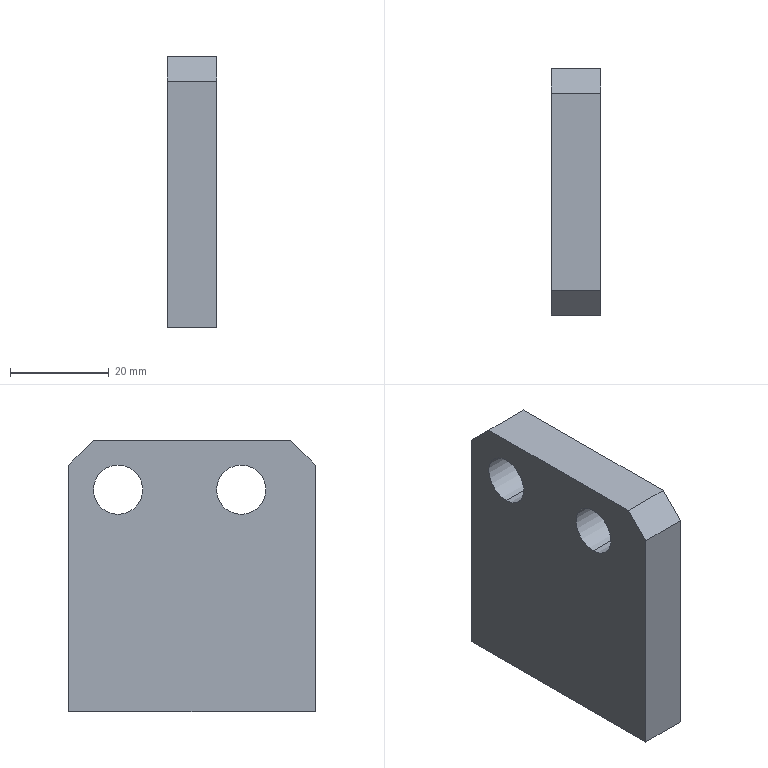Component | SolidWorks | 07-1 | 1 solid | 12 faces | box 10 x 50 x 55 mm | volume 25679 mm3 | plane 8 | cylinder 4 | commonest cylinder face diameters 10 x4
build123d program:
from build123d import *

# Parameters (mm, degrees)
SKETCH1_W           = 55
SKETCH1_H           = 50
SKETCH1_R           = 5
BOSS_EXTRUDE1_DEPTH = 10
CHAMFER1_SIZE       = 5


with BuildPart() as part:
    # Sketch1 → Boss-Extrude1 (new body)
    with BuildSketch(Plane.XY):
        with Locations((-21.5, 205)):
            Rectangle(SKETCH1_W, SKETCH1_H)
        with Locations((-39, 220)):
            Circle(SKETCH1_R, mode=Mode.SUBTRACT)
        with Locations((-39, 195)):
            Circle(SKETCH1_R, mode=Mode.SUBTRACT)
    extrude(amount=BOSS_EXTRUDE1_DEPTH)

    # Chamfer1
    chamfer1_edges = [part.edges().sort_by_distance(p)[0] for p in [
        (-49, 180, 5),
        (-49, 230, 5),
    ]]
    chamfer(chamfer1_edges, length=CHAMFER1_SIZE)


solid = part.part

# Placed as in the assembly
solid = solid.moved(Location((0, 0, 0), (0, 90, 0)))
STEP:
#1=COLOUR_RGB('',0.7922,0.8196,0.9333);
#2=FILL_AREA_STYLE_COLOUR('',#1);
#3=FILL_AREA_STYLE('',(#2));
#4=SURFACE_STYLE_FILL_AREA(#3);
#5=SURFACE_SIDE_STYLE('',(#4));
#6=SURFACE_STYLE_USAGE(.BOTH.,#5);
#7=PRESENTATION_STYLE_ASSIGNMENT((#6));
#8=CARTESIAN_POINT('',(0.3937,7.677,1.732));
#9=VERTEX_POINT('',#8);
#10=CARTESIAN_POINT('',(0.3937,7.677,1.339));
#11=VERTEX_POINT('',#10);
#12=CARTESIAN_POINT('',(0.3937,7.677,1.535));
#13=DIRECTION('',(1.,0.,0.));
#14=DIRECTION('',(0.,0.,-1.));
#15=AXIS2_PLACEMENT_3D('',#12,#13,#14);
#16=CIRCLE('',#15,0.1969);
#17=EDGE_CURVE('',#9,#11,#16,.T.);
#18=ORIENTED_EDGE('',*,*,#17,.T.);
#19=CARTESIAN_POINT('',(0.,7.677,1.339));
#20=VERTEX_POINT('',#19);
#21=CARTESIAN_POINT('',(0.3937,7.677,1.339));
#22=DIRECTION('',(-1.,0.,0.));
#23=VECTOR('',#22,39.37);
#24=LINE('',#21,#23);
#25=EDGE_CURVE('',#11,#20,#24,.T.);
#26=ORIENTED_EDGE('',*,*,#25,.T.);
#27=CARTESIAN_POINT('',(0.,7.677,1.732));
#28=VERTEX_POINT('',#27);
#29=CARTESIAN_POINT('',(0.,7.677,1.535));
#30=DIRECTION('',(1.,0.,0.));
#31=DIRECTION('',(0.,0.,-1.));
#32=AXIS2_PLACEMENT_3D('',#29,#30,#31);
#33=CIRCLE('',#32,0.1969);
#34=EDGE_CURVE('',#28,#20,#33,.T.);
#35=ORIENTED_EDGE('',*,*,#34,.F.);
#36=CARTESIAN_POINT('',(0.3937,7.677,1.732));
#37=DIRECTION('',(-1.,0.,0.));
#38=VECTOR('',#37,39.37);
#39=LINE('',#36,#38);
#40=EDGE_CURVE('',#9,#28,#39,.T.);
#41=ORIENTED_EDGE('',*,*,#40,.F.);
#42=EDGE_LOOP('',(#18,#26,#35,#41));
#43=FACE_OUTER_BOUND('',#42,.T.);
#44=CARTESIAN_POINT('',(0.3937,7.677,1.535));
#45=DIRECTION('',(-1.,0.,0.));
#46=DIRECTION('',(0.,0.,1.));
#47=AXIS2_PLACEMENT_3D('',#44,#45,#46);
#48=CYLINDRICAL_SURFACE('',#47,0.1969);
#49=ADVANCED_FACE('',(#43),#48,.F.);
#50=CARTESIAN_POINT('',(0.3937,8.661,1.732));
#51=VERTEX_POINT('',#50);
#52=CARTESIAN_POINT('',(0.3937,8.661,1.339));
#53=VERTEX_POINT('',#52);
#54=CARTESIAN_POINT('',(0.3937,8.661,1.535));
#55=DIRECTION('',(1.,0.,0.));
#56=DIRECTION('',(0.,0.,-1.));
#57=AXIS2_PLACEMENT_3D('',#54,#55,#56);
#58=CIRCLE('',#57,0.1969);
#59=EDGE_CURVE('',#51,#53,#58,.T.);
#60=ORIENTED_EDGE('',*,*,#59,.T.);
#61=CARTESIAN_POINT('',(0.,8.661,1.339));
#62=VERTEX_POINT('',#61);
#63=CARTESIAN_POINT('',(0.3937,8.661,1.339));
#64=DIRECTION('',(-1.,0.,0.));
#65=VECTOR('',#64,39.37);
#66=LINE('',#63,#65);
#67=EDGE_CURVE('',#53,#62,#66,.T.);
#68=ORIENTED_EDGE('',*,*,#67,.T.);
#69=CARTESIAN_POINT('',(0.,8.661,1.732));
#70=VERTEX_POINT('',#69);
#71=CARTESIAN_POINT('',(0.,8.661,1.535));
#72=DIRECTION('',(1.,0.,0.));
#73=DIRECTION('',(0.,0.,-1.));
#74=AXIS2_PLACEMENT_3D('',#71,#72,#73);
#75=CIRCLE('',#74,0.1969);
#76=EDGE_CURVE('',#70,#62,#75,.T.);
#77=ORIENTED_EDGE('',*,*,#76,.F.);
#78=CARTESIAN_POINT('',(0.3937,8.661,1.732));
#79=DIRECTION('',(-1.,0.,0.));
#80=VECTOR('',#79,39.37);
#81=LINE('',#78,#80);
#82=EDGE_CURVE('',#51,#70,#81,.T.);
#83=ORIENTED_EDGE('',*,*,#82,.F.);
#84=EDGE_LOOP('',(#60,#68,#77,#83));
#85=FACE_OUTER_BOUND('',#84,.T.);
#86=CARTESIAN_POINT('',(0.3937,8.661,1.535));
#87=DIRECTION('',(-1.,0.,0.));
#88=DIRECTION('',(0.,0.,1.));
#89=AXIS2_PLACEMENT_3D('',#86,#87,#88);
#90=CYLINDRICAL_SURFACE('',#89,0.1969);
#91=ADVANCED_FACE('',(#85),#90,.F.);
#92=CARTESIAN_POINT('',(0.3937,8.858,1.929));
#93=VERTEX_POINT('',#92);
#94=CARTESIAN_POINT('',(0.3937,7.283,1.929));
#95=VERTEX_POINT('',#94);
#96=CARTESIAN_POINT('',(0.3937,9.055,1.929));
#97=DIRECTION('',(0.,-1.,-0.));
#98=VECTOR('',#97,39.37);
#99=LINE('',#96,#98);
#100=EDGE_CURVE('',#93,#95,#99,.T.);
#101=ORIENTED_EDGE('',*,*,#100,.T.);
#102=CARTESIAN_POINT('',(0.3937,7.087,1.732));
#103=VERTEX_POINT('',#102);
#104=CARTESIAN_POINT('',(0.3937,7.087,1.732));
#105=DIRECTION('',(0.,-0.7071,-0.7071));
#106=VECTOR('',#105,39.37);
#107=LINE('',#104,#106);
#108=EDGE_CURVE('',#95,#103,#107,.T.);
#109=ORIENTED_EDGE('',*,*,#108,.T.);
#110=CARTESIAN_POINT('',(0.3937,7.087,-0.2362));
#111=VERTEX_POINT('',#110);
#112=CARTESIAN_POINT('',(0.3937,7.087,-0.2362));
#113=DIRECTION('',(0.,0.,-1.));
#114=VECTOR('',#113,39.37);
#115=LINE('',#112,#114);
#116=EDGE_CURVE('',#103,#111,#115,.T.);
#117=ORIENTED_EDGE('',*,*,#116,.T.);
#118=CARTESIAN_POINT('',(0.3937,9.055,-0.2362));
#119=VERTEX_POINT('',#118);
#120=CARTESIAN_POINT('',(0.3937,9.055,-0.2362));
#121=DIRECTION('',(0.,1.,0.));
#122=VECTOR('',#121,39.37);
#123=LINE('',#120,#122);
#124=EDGE_CURVE('',#111,#119,#123,.T.);
#125=ORIENTED_EDGE('',*,*,#124,.T.);
#126=CARTESIAN_POINT('',(0.3937,9.055,1.732));
#127=VERTEX_POINT('',#126);
#128=CARTESIAN_POINT('',(0.3937,9.055,-0.2362));
#129=DIRECTION('',(0.,0.,1.));
#130=VECTOR('',#129,39.37);
#131=LINE('',#128,#130);
#132=EDGE_CURVE('',#119,#127,#131,.T.);
#133=ORIENTED_EDGE('',*,*,#132,.T.);
#134=CARTESIAN_POINT('',(0.3937,8.858,1.929));
#135=DIRECTION('',(0.,-0.7071,0.7071));
#136=VECTOR('',#135,39.37);
#137=LINE('',#134,#136);
#138=EDGE_CURVE('',#127,#93,#137,.T.);
#139=ORIENTED_EDGE('',*,*,#138,.T.);
#140=EDGE_LOOP('',(#101,#109,#117,#125,#133,#139));
#141=FACE_OUTER_BOUND('',#140,.T.);
#142=ORIENTED_EDGE('',*,*,#59,.F.);
#143=CARTESIAN_POINT('',(0.3937,8.661,1.535));
#144=DIRECTION('',(1.,0.,0.));
#145=DIRECTION('',(0.,0.,-1.));
#146=AXIS2_PLACEMENT_3D('',#143,#144,#145);
#147=CIRCLE('',#146,0.1969);
#148=EDGE_CURVE('',#53,#51,#147,.T.);
#149=ORIENTED_EDGE('',*,*,#148,.F.);
#150=EDGE_LOOP('',(#142,#149));
#151=FACE_BOUND('',#150,.T.);
#152=ORIENTED_EDGE('',*,*,#17,.F.);
#153=CARTESIAN_POINT('',(0.3937,7.677,1.535));
#154=DIRECTION('',(1.,0.,0.));
#155=DIRECTION('',(0.,0.,-1.));
#156=AXIS2_PLACEMENT_3D('',#153,#154,#155);
#157=CIRCLE('',#156,0.1969);
#158=EDGE_CURVE('',#11,#9,#157,.T.);
#159=ORIENTED_EDGE('',*,*,#158,.F.);
#160=EDGE_LOOP('',(#152,#159));
#161=FACE_BOUND('',#160,.T.);
#162=CARTESIAN_POINT('',(0.3937,0.,0.));
#163=DIRECTION('',(-1.,0.,0.));
#164=DIRECTION('',(0.,0.,1.));
#165=AXIS2_PLACEMENT_3D('',#162,#163,#164);
#166=PLANE('',#165);
#167=ADVANCED_FACE('',(#141,#151,#161),#166,.F.);
#168=ORIENTED_EDGE('',*,*,#76,.T.);
#169=CARTESIAN_POINT('',(0.,8.661,1.535));
#170=DIRECTION('',(1.,0.,0.));
#171=DIRECTION('',(0.,0.,-1.));
#172=AXIS2_PLACEMENT_3D('',#169,#170,#171);
#173=CIRCLE('',#172,0.1969);
#174=EDGE_CURVE('',#62,#70,#173,.T.);
#175=ORIENTED_EDGE('',*,*,#174,.T.);
#176=EDGE_LOOP('',(#168,#175));
#177=FACE_BOUND('',#176,.T.);
#178=CARTESIAN_POINT('',(0.,7.087,1.732));
#179=VERTEX_POINT('',#178);
#180=CARTESIAN_POINT('',(0.,7.087,-0.2362));
#181=VERTEX_POINT('',#180);
#182=CARTESIAN_POINT('',(0.,7.087,-0.2362));
#183=DIRECTION('',(0.,0.,-1.));
#184=VECTOR('',#183,39.37);
#185=LINE('',#182,#184);
#186=EDGE_CURVE('',#179,#181,#185,.T.);
#187=ORIENTED_EDGE('',*,*,#186,.F.);
#188=CARTESIAN_POINT('',(0.,7.283,1.929));
#189=VERTEX_POINT('',#188);
#190=CARTESIAN_POINT('',(0.,2.677,-2.677));
#191=DIRECTION('',(0.,0.7071,0.7071));
#192=VECTOR('',#191,39.37);
#193=LINE('',#190,#192);
#194=EDGE_CURVE('',#179,#189,#193,.T.);
#195=ORIENTED_EDGE('',*,*,#194,.T.);
#196=CARTESIAN_POINT('',(0.,8.858,1.929));
#197=VERTEX_POINT('',#196);
#198=CARTESIAN_POINT('',(0.,9.055,1.929));
#199=DIRECTION('',(0.,-1.,-0.));
#200=VECTOR('',#199,39.37);
#201=LINE('',#198,#200);
#202=EDGE_CURVE('',#197,#189,#201,.T.);
#203=ORIENTED_EDGE('',*,*,#202,.F.);
#204=CARTESIAN_POINT('',(0.,9.055,1.732));
#205=VERTEX_POINT('',#204);
#206=CARTESIAN_POINT('',(0.,5.394,5.394));
#207=DIRECTION('',(0.,0.7071,-0.7071));
#208=VECTOR('',#207,39.37);
#209=LINE('',#206,#208);
#210=EDGE_CURVE('',#197,#205,#209,.T.);
#211=ORIENTED_EDGE('',*,*,#210,.T.);
#212=CARTESIAN_POINT('',(0.,9.055,-0.2362));
#213=VERTEX_POINT('',#212);
#214=CARTESIAN_POINT('',(0.,9.055,-0.2362));
#215=DIRECTION('',(0.,0.,1.));
#216=VECTOR('',#215,39.37);
#217=LINE('',#214,#216);
#218=EDGE_CURVE('',#213,#205,#217,.T.);
#219=ORIENTED_EDGE('',*,*,#218,.F.);
#220=CARTESIAN_POINT('',(0.,9.055,-0.2362));
#221=DIRECTION('',(0.,1.,0.));
#222=VECTOR('',#221,39.37);
#223=LINE('',#220,#222);
#224=EDGE_CURVE('',#181,#213,#223,.T.);
#225=ORIENTED_EDGE('',*,*,#224,.F.);
#226=EDGE_LOOP('',(#187,#195,#203,#211,#219,#225));
#227=FACE_OUTER_BOUND('',#226,.T.);
#228=ORIENTED_EDGE('',*,*,#34,.T.);
#229=CARTESIAN_POINT('',(0.,7.677,1.535));
#230=DIRECTION('',(1.,0.,0.));
#231=DIRECTION('',(0.,0.,-1.));
#232=AXIS2_PLACEMENT_3D('',#229,#230,#231);
#233=CIRCLE('',#232,0.1969);
#234=EDGE_CURVE('',#20,#28,#233,.T.);
#235=ORIENTED_EDGE('',*,*,#234,.T.);
#236=EDGE_LOOP('',(#228,#235));
#237=FACE_BOUND('',#236,.T.);
#238=CARTESIAN_POINT('',(0.,0.,0.));
#239=DIRECTION('',(-1.,0.,0.));
#240=DIRECTION('',(0.,0.,1.));
#241=AXIS2_PLACEMENT_3D('',#238,#239,#240);
#242=PLANE('',#241);
#243=ADVANCED_FACE('',(#177,#227,#237),#242,.T.);
#244=ORIENTED_EDGE('',*,*,#224,.T.);
#245=CARTESIAN_POINT('',(0.3937,9.055,-0.2362));
#246=DIRECTION('',(-1.,0.,0.));
#247=VECTOR('',#246,39.37);
#248=LINE('',#245,#247);
#249=EDGE_CURVE('',#119,#213,#248,.T.);
#250=ORIENTED_EDGE('',*,*,#249,.F.);
#251=ORIENTED_EDGE('',*,*,#124,.F.);
#252=CARTESIAN_POINT('',(0.3937,7.087,-0.2362));
#253=DIRECTION('',(-1.,0.,0.));
#254=VECTOR('',#253,39.37);
#255=LINE('',#252,#254);
#256=EDGE_CURVE('',#111,#181,#255,.T.);
#257=ORIENTED_EDGE('',*,*,#256,.T.);
#258=EDGE_LOOP('',(#244,#250,#251,#257));
#259=FACE_OUTER_BOUND('',#258,.T.);
#260=CARTESIAN_POINT('',(0.3937,9.055,-0.2362));
#261=DIRECTION('',(0.,-0.,1.));
#262=DIRECTION('',(0.,-1.,-0.));
#263=AXIS2_PLACEMENT_3D('',#260,#261,#262);
#264=PLANE('',#263);
#265=ADVANCED_FACE('',(#259),#264,.F.);
#266=ORIENTED_EDGE('',*,*,#218,.T.);
#267=CARTESIAN_POINT('',(0.3937,9.055,1.732));
#268=DIRECTION('',(1.,0.,0.));
#269=VECTOR('',#268,39.37);
#270=LINE('',#267,#269);
#271=EDGE_CURVE('',#205,#127,#270,.T.);
#272=ORIENTED_EDGE('',*,*,#271,.T.);
#273=ORIENTED_EDGE('',*,*,#132,.F.);
#274=ORIENTED_EDGE('',*,*,#249,.T.);
#275=EDGE_LOOP('',(#266,#272,#273,#274));
#276=FACE_OUTER_BOUND('',#275,.T.);
#277=CARTESIAN_POINT('',(0.3937,9.055,-0.2362));
#278=DIRECTION('',(0.,-1.,0.));
#279=DIRECTION('',(0.,-0.,-1.));
#280=AXIS2_PLACEMENT_3D('',#277,#278,#279);
#281=PLANE('',#280);
#282=ADVANCED_FACE('',(#276),#281,.F.);
#283=ORIENTED_EDGE('',*,*,#202,.T.);
#284=CARTESIAN_POINT('',(0.3937,7.283,1.929));
#285=DIRECTION('',(1.,0.,0.));
#286=VECTOR('',#285,39.37);
#287=LINE('',#284,#286);
#288=EDGE_CURVE('',#189,#95,#287,.T.);
#289=ORIENTED_EDGE('',*,*,#288,.T.);
#290=ORIENTED_EDGE('',*,*,#100,.F.);
#291=CARTESIAN_POINT('',(0.3937,8.858,1.929));
#292=DIRECTION('',(-1.,0.,0.));
#293=VECTOR('',#292,39.37);
#294=LINE('',#291,#293);
#295=EDGE_CURVE('',#93,#197,#294,.T.);
#296=ORIENTED_EDGE('',*,*,#295,.T.);
#297=EDGE_LOOP('',(#283,#289,#290,#296));
#298=FACE_OUTER_BOUND('',#297,.T.);
#299=CARTESIAN_POINT('',(0.3937,9.055,1.929));
#300=DIRECTION('',(0.,0.,-1.));
#301=DIRECTION('',(0.,1.,0.));
#302=AXIS2_PLACEMENT_3D('',#299,#300,#301);
#303=PLANE('',#302);
#304=ADVANCED_FACE('',(#298),#303,.F.);
#305=ORIENTED_EDGE('',*,*,#116,.F.);
#306=CARTESIAN_POINT('',(0.3937,7.087,1.732));
#307=DIRECTION('',(-1.,0.,0.));
#308=VECTOR('',#307,39.37);
#309=LINE('',#306,#308);
#310=EDGE_CURVE('',#103,#179,#309,.T.);
#311=ORIENTED_EDGE('',*,*,#310,.T.);
#312=ORIENTED_EDGE('',*,*,#186,.T.);
#313=ORIENTED_EDGE('',*,*,#256,.F.);
#314=EDGE_LOOP('',(#305,#311,#312,#313));
#315=FACE_OUTER_BOUND('',#314,.T.);
#316=CARTESIAN_POINT('',(0.3937,7.087,-0.2362));
#317=DIRECTION('',(0.,1.,0.));
#318=DIRECTION('',(1.,0.,0.));
#319=AXIS2_PLACEMENT_3D('',#316,#317,#318);
#320=PLANE('',#319);
#321=ADVANCED_FACE('',(#315),#320,.F.);
#322=ORIENTED_EDGE('',*,*,#67,.F.);
#323=ORIENTED_EDGE('',*,*,#148,.T.);
#324=ORIENTED_EDGE('',*,*,#82,.T.);
#325=ORIENTED_EDGE('',*,*,#174,.F.);
#326=EDGE_LOOP('',(#322,#323,#324,#325));
#327=FACE_OUTER_BOUND('',#326,.T.);
#328=CARTESIAN_POINT('',(0.3937,8.661,1.535));
#329=DIRECTION('',(-1.,0.,0.));
#330=DIRECTION('',(0.,0.,1.));
#331=AXIS2_PLACEMENT_3D('',#328,#329,#330);
#332=CYLINDRICAL_SURFACE('',#331,0.1969);
#333=ADVANCED_FACE('',(#327),#332,.F.);
#334=ORIENTED_EDGE('',*,*,#25,.F.);
#335=ORIENTED_EDGE('',*,*,#158,.T.);
#336=ORIENTED_EDGE('',*,*,#40,.T.);
#337=ORIENTED_EDGE('',*,*,#234,.F.);
#338=EDGE_LOOP('',(#334,#335,#336,#337));
#339=FACE_OUTER_BOUND('',#338,.T.);
#340=CARTESIAN_POINT('',(0.3937,7.677,1.535));
#341=DIRECTION('',(-1.,0.,0.));
#342=DIRECTION('',(0.,0.,1.));
#343=AXIS2_PLACEMENT_3D('',#340,#341,#342);
#344=CYLINDRICAL_SURFACE('',#343,0.1969);
#345=ADVANCED_FACE('',(#339),#344,.F.);
#346=ORIENTED_EDGE('',*,*,#108,.F.);
#347=ORIENTED_EDGE('',*,*,#288,.F.);
#348=ORIENTED_EDGE('',*,*,#194,.F.);
#349=ORIENTED_EDGE('',*,*,#310,.F.);
#350=EDGE_LOOP('',(#346,#347,#348,#349));
#351=FACE_OUTER_BOUND('',#350,.T.);
#352=CARTESIAN_POINT('',(0.3937,7.087,1.732));
#353=DIRECTION('',(0.,0.7071,-0.7071));
#354=DIRECTION('',(-1.,0.,0.));
#355=AXIS2_PLACEMENT_3D('',#352,#353,#354);
#356=PLANE('',#355);
#357=ADVANCED_FACE('',(#351),#356,.F.);
#358=ORIENTED_EDGE('',*,*,#138,.F.);
#359=ORIENTED_EDGE('',*,*,#271,.F.);
#360=ORIENTED_EDGE('',*,*,#210,.F.);
#361=ORIENTED_EDGE('',*,*,#295,.F.);
#362=EDGE_LOOP('',(#358,#359,#360,#361));
#363=FACE_OUTER_BOUND('',#362,.T.);
#364=CARTESIAN_POINT('',(0.3937,8.858,1.929));
#365=DIRECTION('',(0.,-0.7071,-0.7071));
#366=DIRECTION('',(-1.,0.,0.));
#367=AXIS2_PLACEMENT_3D('',#364,#365,#366);
#368=PLANE('',#367);
#369=ADVANCED_FACE('',(#363),#368,.F.);
#370=CLOSED_SHELL('',(#49,#91,#167,#243,#265,#282,#304,#321,#333,#345,#357,#369));
#371=MANIFOLD_SOLID_BREP('',#370);
#372=STYLED_ITEM('',(#7),#371);
#373=PRESENTATION_LAYER_ASSIGNMENT('','',(#372));
#374=CARTESIAN_POINT('',(0.,0.,0.));
#375=DIRECTION('',(0.,0.,1.));
#376=DIRECTION('',(1.,0.,0.));
#377=AXIS2_PLACEMENT_3D('',#374,#375,#376);
#378=(LENGTH_UNIT()NAMED_UNIT(*)SI_UNIT($,.METRE.));
#379=LENGTH_MEASURE_WITH_UNIT(LENGTH_MEASURE(0.0254),#378);
#380=DIMENSIONAL_EXPONENTS(1.,0.,0.,0.,0.,0.,0.);
#381=(CONVERSION_BASED_UNIT('',#379)LENGTH_UNIT()NAMED_UNIT(#380));
#382=UNCERTAINTY_MEASURE_WITH_UNIT(LENGTH_MEASURE(0.00001),#381,'','');
#383=(NAMED_UNIT(*)PLANE_ANGLE_UNIT()SI_UNIT($,.RADIAN.));
#384=(NAMED_UNIT(*)SI_UNIT($,.STERADIAN.)SOLID_ANGLE_UNIT());
#385=(GEOMETRIC_REPRESENTATION_CONTEXT(3)GLOBAL_UNCERTAINTY_ASSIGNED_CONTEXT((#382))GLOBAL_UNIT_ASSIGNED_CONTEXT((#381,#383,#384))REPRESENTATION_CONTEXT('',''));
#386=ADVANCED_BREP_SHAPE_REPRESENTATION('',(#371,#377),#385);
#387=(LENGTH_UNIT()NAMED_UNIT(*)SI_UNIT($,.METRE.));
#388=LENGTH_MEASURE_WITH_UNIT(LENGTH_MEASURE(0.0254),#387);
#389=DIMENSIONAL_EXPONENTS(1.,0.,0.,0.,0.,0.,0.);
#390=(CONVERSION_BASED_UNIT('',#388)LENGTH_UNIT()NAMED_UNIT(#389));
#391=UNCERTAINTY_MEASURE_WITH_UNIT(LENGTH_MEASURE(0.00001),#390,'','');
#392=(NAMED_UNIT(*)PLANE_ANGLE_UNIT()SI_UNIT($,.RADIAN.));
#393=(NAMED_UNIT(*)SI_UNIT($,.STERADIAN.)SOLID_ANGLE_UNIT());
#394=(GEOMETRIC_REPRESENTATION_CONTEXT(3)GLOBAL_UNCERTAINTY_ASSIGNED_CONTEXT((#391))GLOBAL_UNIT_ASSIGNED_CONTEXT((#390,#392,#393))REPRESENTATION_CONTEXT('',''));
#395=MECHANICAL_DESIGN_GEOMETRIC_PRESENTATION_REPRESENTATION('',(#372),#394);